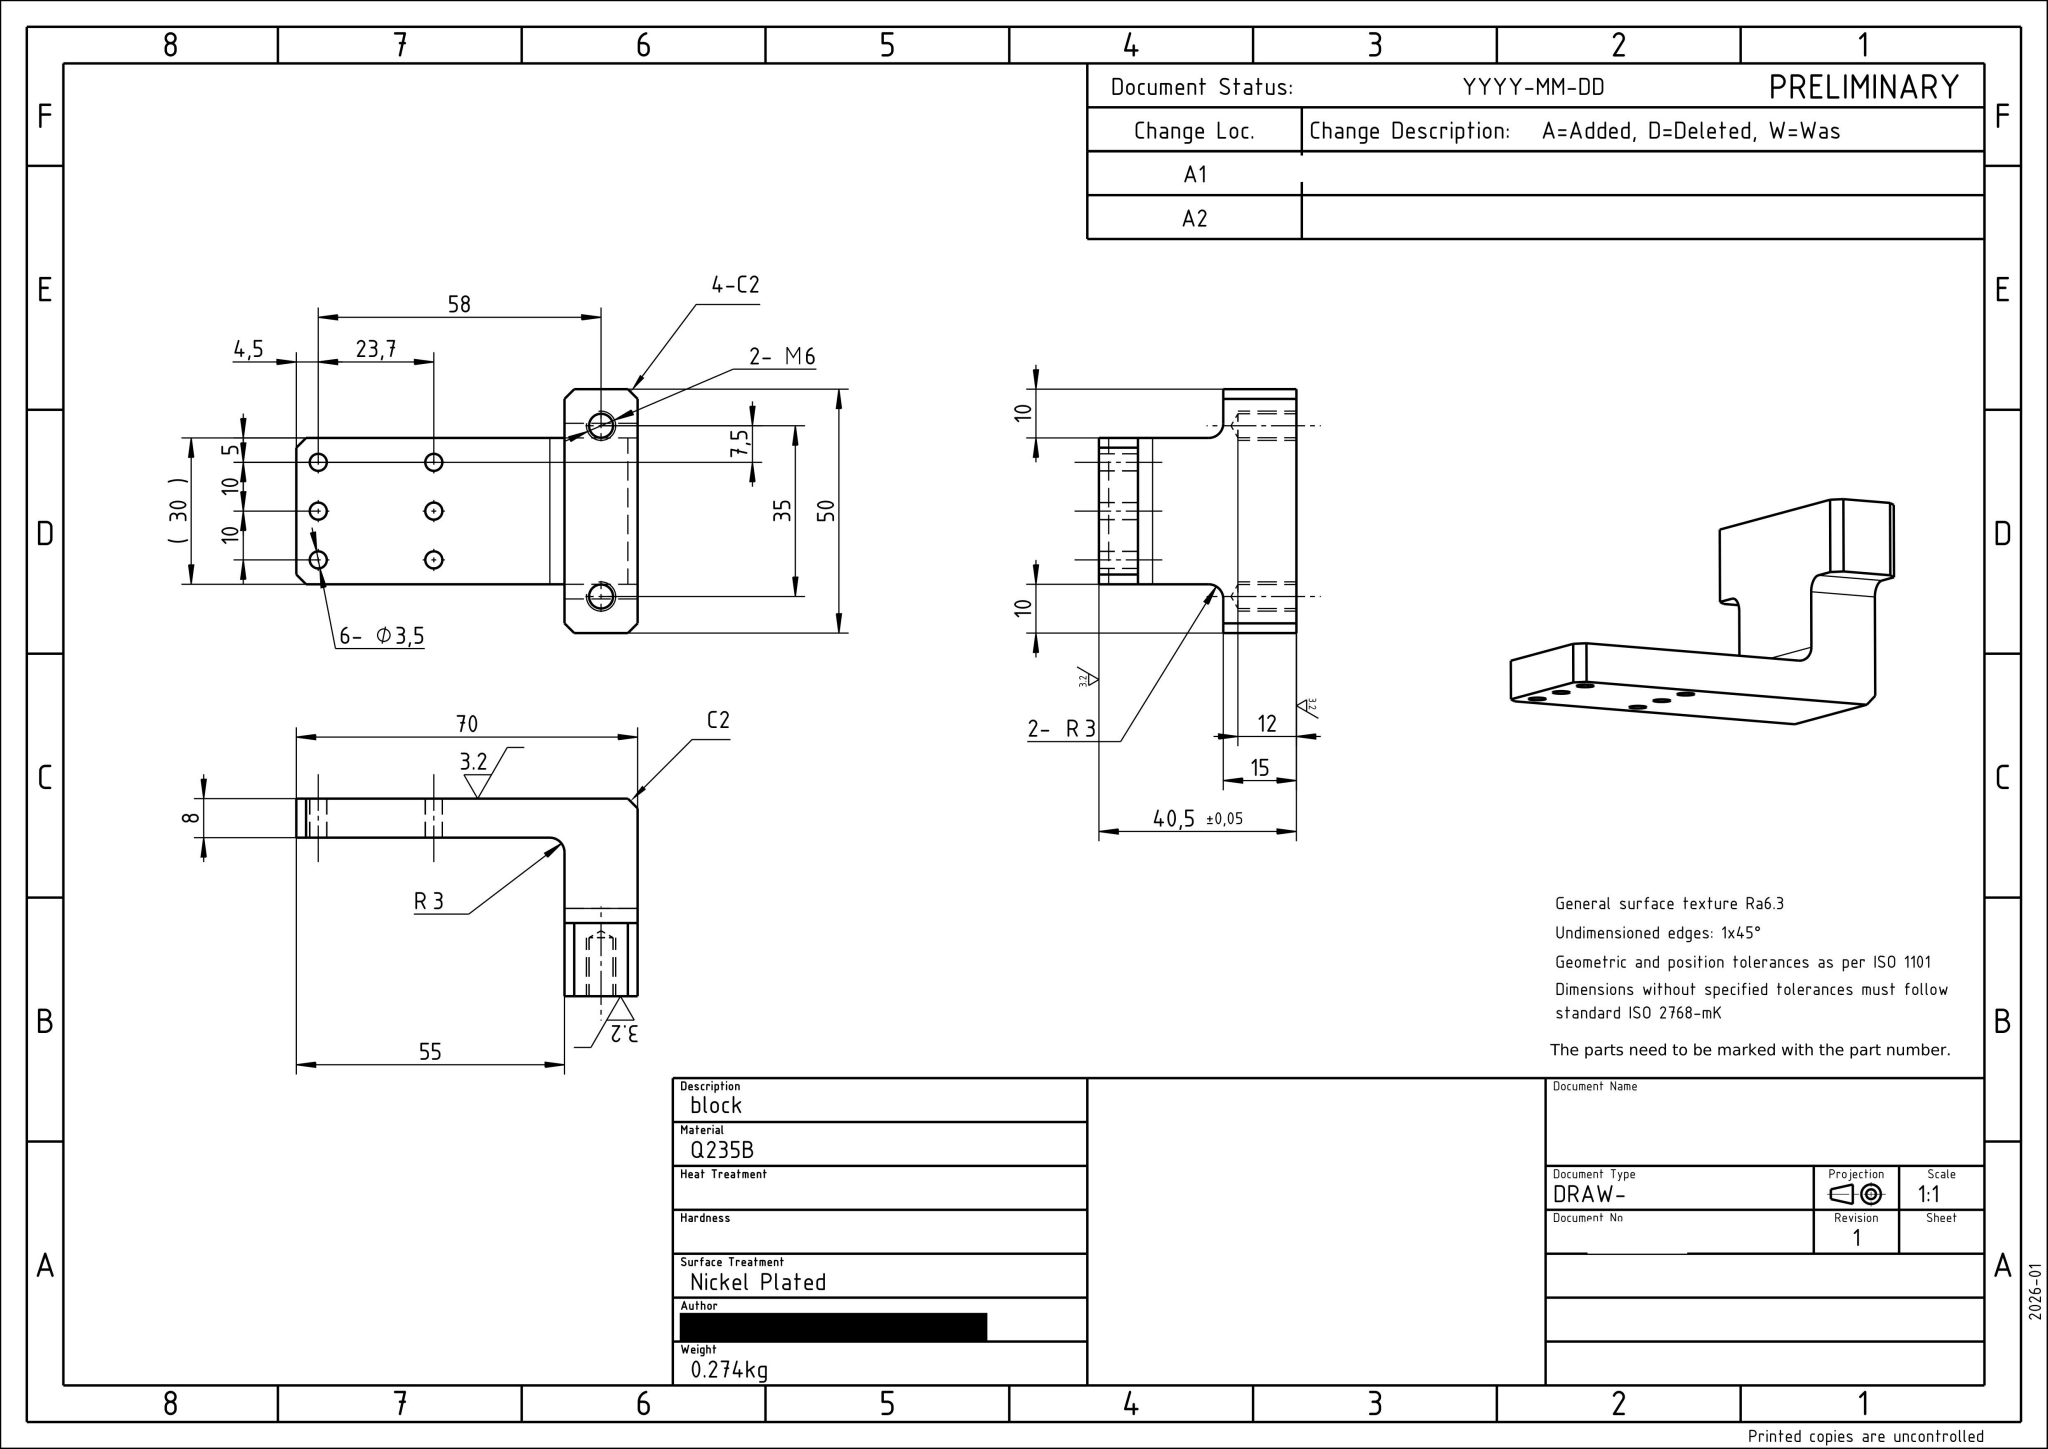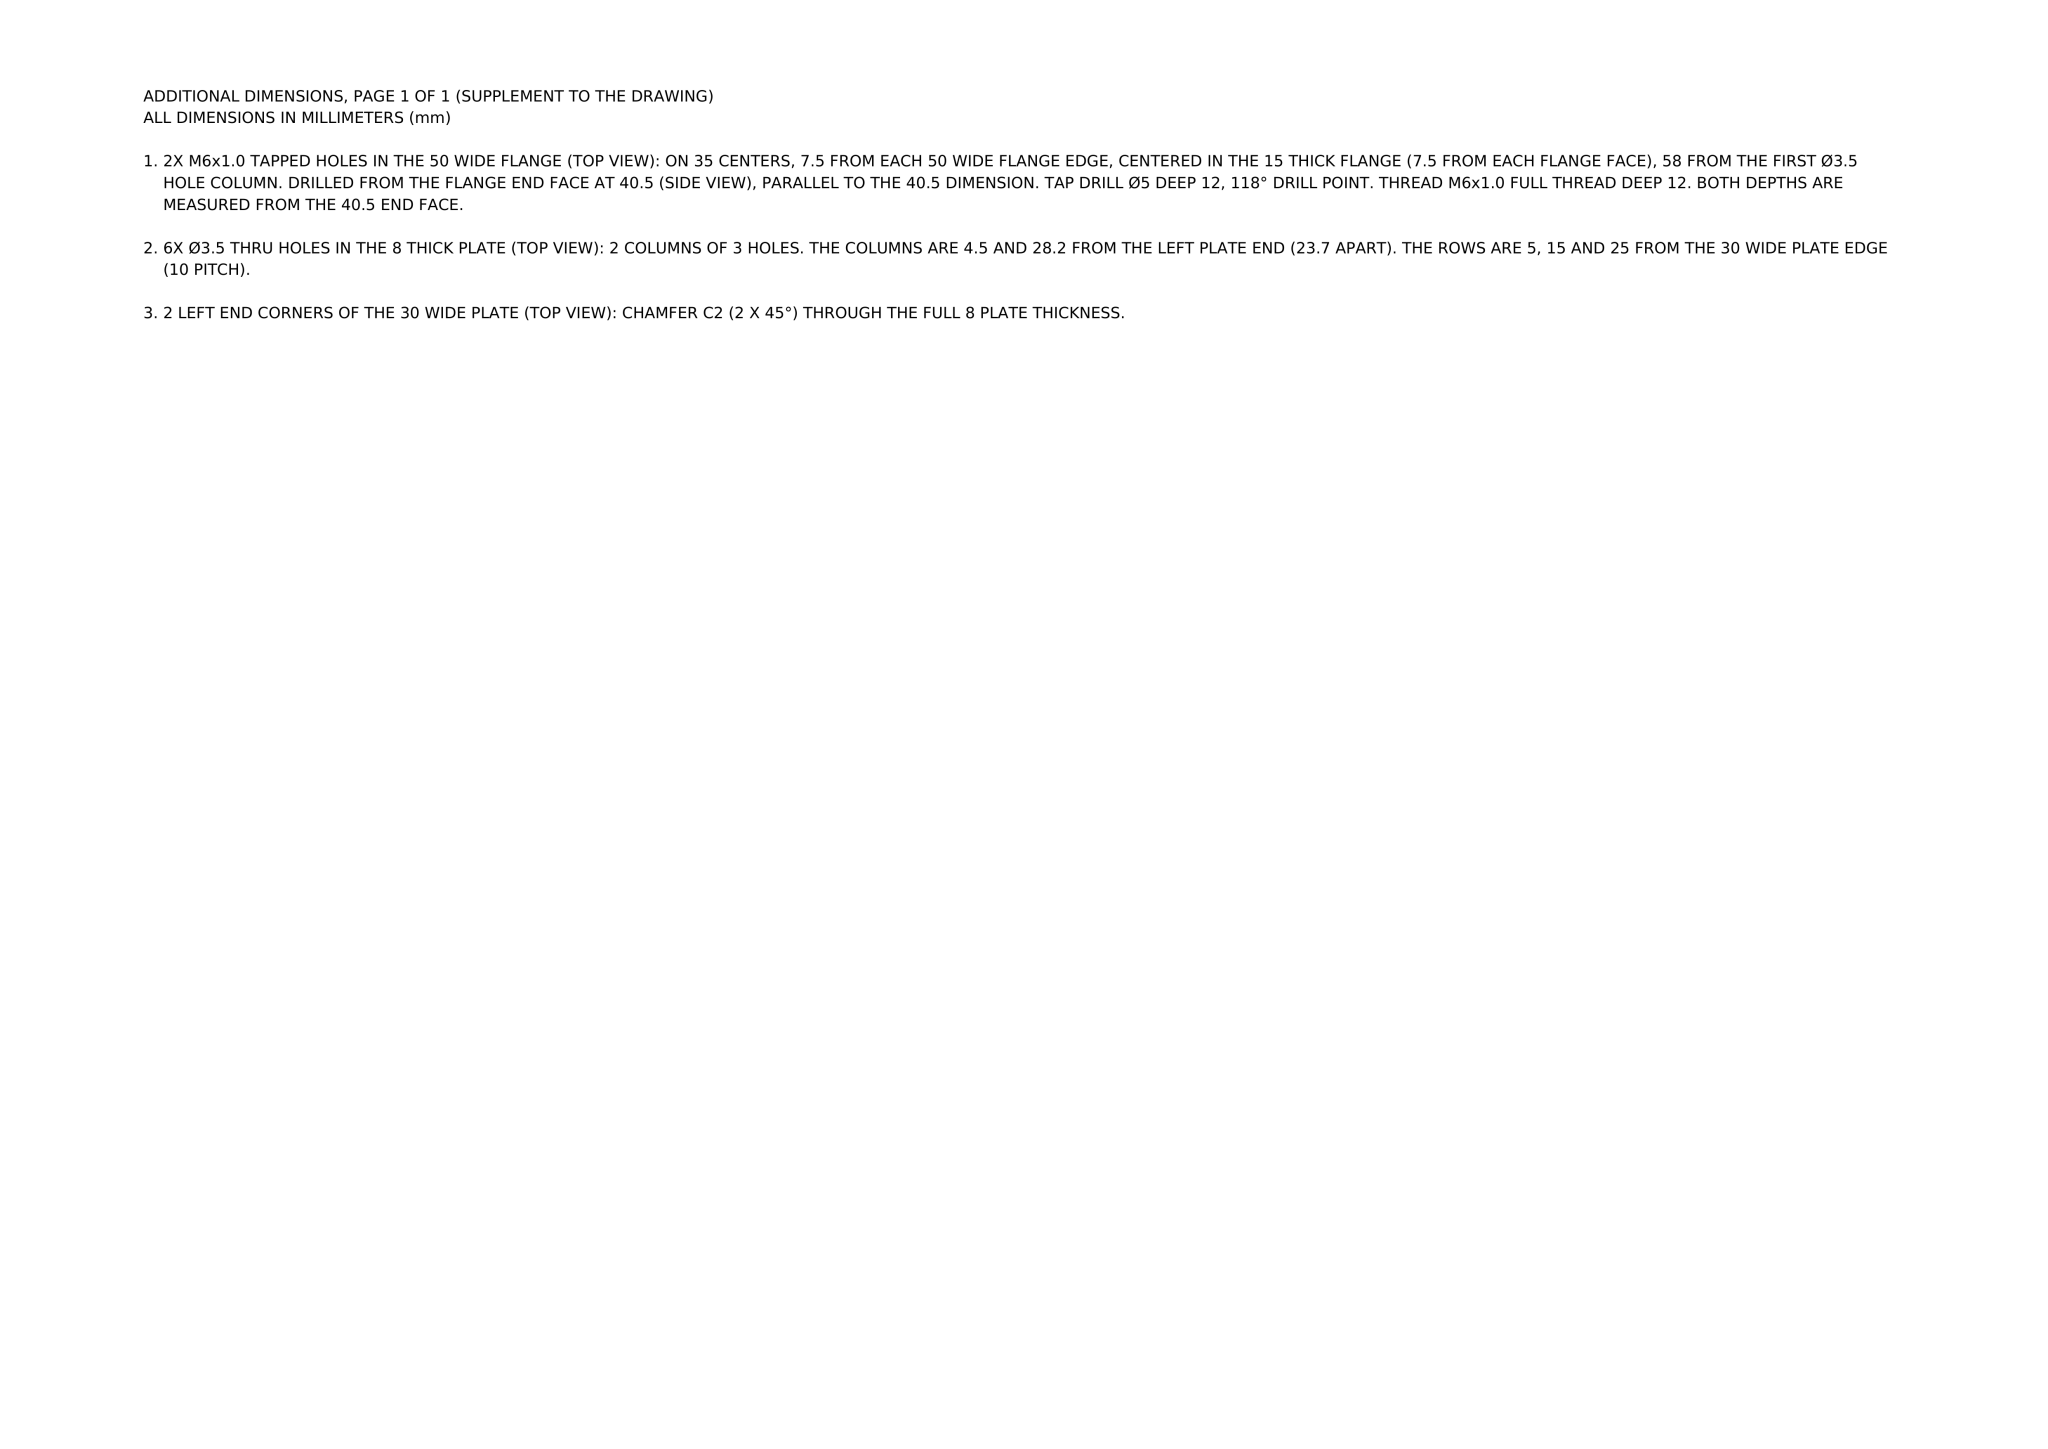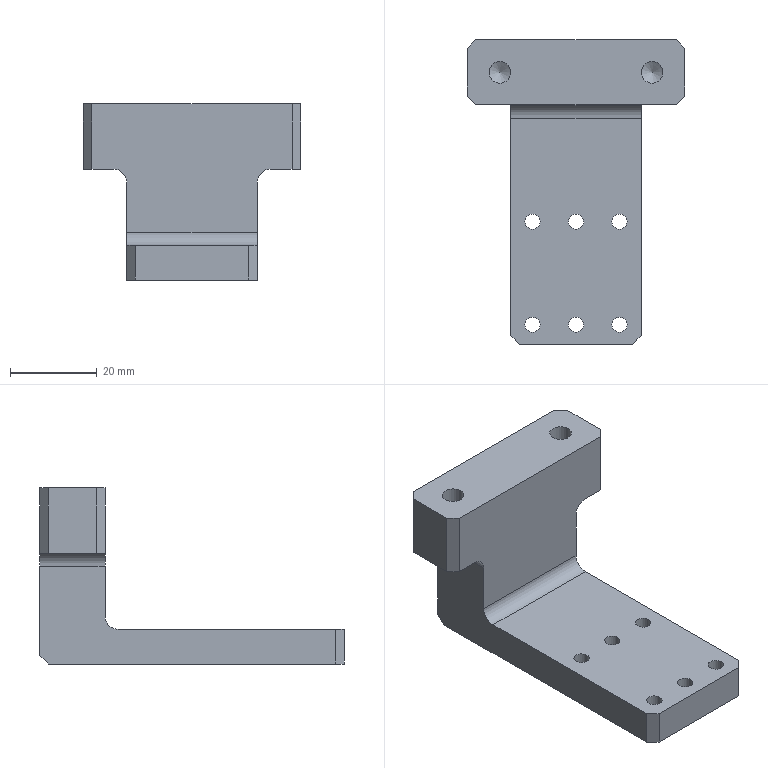Part | NX | mm | 1 solid | 32 faces | box 50 x 70 x 40.5 mm | volume 34876 mm3 | plane 19 | cylinder 11 | cone 2 | commonest cylinder face diameters 3.5 x6 6 x3 5 x2